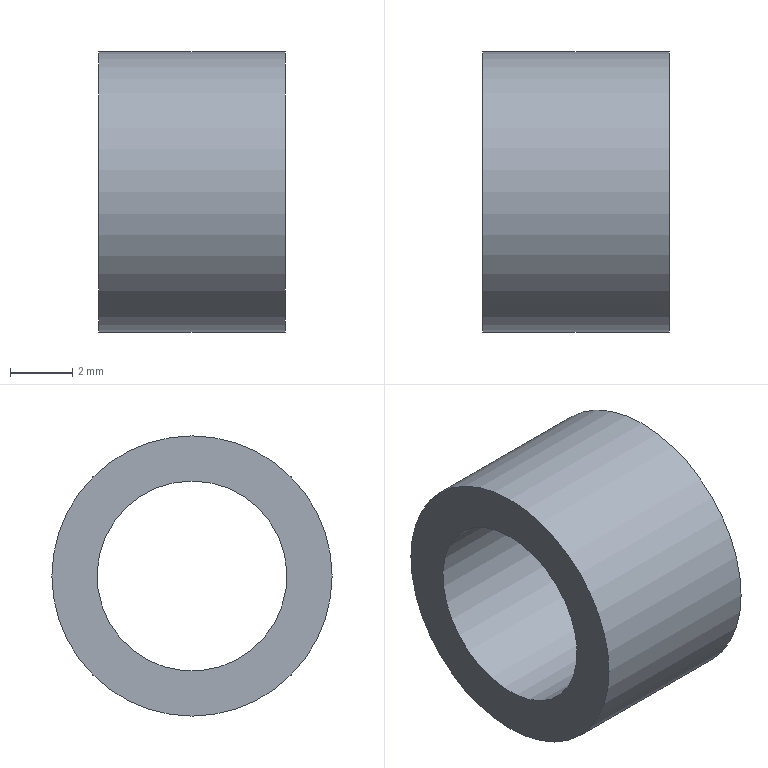Component | NX | BUSHING | 1 solid | 4 faces | box 6 x 9 x 9 mm | volume 206 mm3 | cylinder 2 | plane 2 | commonest cylinder face diameters 9 x1 6.1 x1
STEP:
#1=CARTESIAN_POINT('',(0.,0.,0.));
#2=DIRECTION('',(0.,0.,1.));
#3=DIRECTION('',(1.,0.,0.));
#4=AXIS2_PLACEMENT_3D('',#1,#2,#3);
#5=CARTESIAN_POINT('',(15.144,16.19,-72.915));
#6=VERTEX_POINT('',#5);
#7=CARTESIAN_POINT('',(15.144,16.19,-77.415));
#8=DIRECTION('',(-1.,0.,0.));
#9=DIRECTION('',(0.,0.,1.));
#10=AXIS2_PLACEMENT_3D('',#7,#8,#9);
#11=CIRCLE('',#10,4.5);
#12=CARTESIAN_POINT('',(15.144,16.19,-77.415));
#13=DIRECTION('',(1.,0.,0.));
#14=DIRECTION('',(0.,0.,-1.));
#15=AXIS2_PLACEMENT_3D('',#12,#13,#14);
#16=CYLINDRICAL_SURFACE('',#15,4.5);
#17=CARTESIAN_POINT('',(9.425,0.));
#18=DIRECTION('',(-1.,0.));
#19=VECTOR('',#18,1.);
#20=LINE('',#17,#19);
#21=(GEOMETRIC_REPRESENTATION_CONTEXT(2)PARAMETRIC_REPRESENTATION_CONTEXT()REPRESENTATION_CONTEXT('',''));
#22=DEFINITIONAL_REPRESENTATION('',(#20),#21);
#23=PCURVE('',#16,#22);
#24=CARTESIAN_POINT('',(15.144,16.19,-77.415));
#25=DIRECTION('',(-1.,0.,0.));
#26=DIRECTION('',(0.,0.,1.));
#27=AXIS2_PLACEMENT_3D('',#24,#25,#26);
#28=PLANE('',#27);
#29=CARTESIAN_POINT('',(0.,0.));
#30=DIRECTION('',(1.,0.));
#31=AXIS2_PLACEMENT_2D('',#29,#30);
#32=CIRCLE('',#31,4.5);
#33=(GEOMETRIC_REPRESENTATION_CONTEXT(2)PARAMETRIC_REPRESENTATION_CONTEXT()REPRESENTATION_CONTEXT('',''));
#34=DEFINITIONAL_REPRESENTATION('',(#32),#33);
#35=PCURVE('',#28,#34);
#36=SURFACE_CURVE('',#11,(#23,#35),.PCURVE_S1.);
#37=EDGE_CURVE('',#6,#6,#36,.T.);
#38=ORIENTED_EDGE('',*,*,#37,.F.);
#39=CARTESIAN_POINT('',(21.144,16.19,-72.915));
#40=VERTEX_POINT('',#39);
#41=CARTESIAN_POINT('',(15.144,16.19,-72.915));
#42=CARTESIAN_POINT('',(21.144,16.19,-72.915));
#43=B_SPLINE_CURVE_WITH_KNOTS('',1,(#41,#42),.UNSPECIFIED.,.F.,.F.,(2,2),(0.,6.),.PIECEWISE_BEZIER_KNOTS.);
#44=CARTESIAN_POINT('',(9.425,0.));
#45=DIRECTION('',(0.,1.));
#46=VECTOR('',#45,1.);
#47=LINE('',#44,#46);
#48=(GEOMETRIC_REPRESENTATION_CONTEXT(2)PARAMETRIC_REPRESENTATION_CONTEXT()REPRESENTATION_CONTEXT('',''));
#49=DEFINITIONAL_REPRESENTATION('',(#47),#48);
#50=PCURVE('',#16,#49);
#51=CARTESIAN_POINT('',(3.142,0.));
#52=DIRECTION('',(0.,1.));
#53=VECTOR('',#52,1.);
#54=LINE('',#51,#53);
#55=(GEOMETRIC_REPRESENTATION_CONTEXT(2)PARAMETRIC_REPRESENTATION_CONTEXT()REPRESENTATION_CONTEXT('',''));
#56=DEFINITIONAL_REPRESENTATION('',(#54),#55);
#57=PCURVE('',#16,#56);
#58=SEAM_CURVE('',#43,(#50,#57),.PCURVE_S1.);
#59=EDGE_CURVE('',#6,#40,#58,.T.);
#60=ORIENTED_EDGE('',*,*,#59,.T.);
#61=CARTESIAN_POINT('',(21.144,16.19,-77.415));
#62=DIRECTION('',(-1.,0.,0.));
#63=DIRECTION('',(0.,0.,1.));
#64=AXIS2_PLACEMENT_3D('',#61,#62,#63);
#65=CIRCLE('',#64,4.5);
#66=CARTESIAN_POINT('',(9.425,6.));
#67=DIRECTION('',(-1.,0.));
#68=VECTOR('',#67,1.);
#69=LINE('',#66,#68);
#70=(GEOMETRIC_REPRESENTATION_CONTEXT(2)PARAMETRIC_REPRESENTATION_CONTEXT()REPRESENTATION_CONTEXT('',''));
#71=DEFINITIONAL_REPRESENTATION('',(#69),#70);
#72=PCURVE('',#16,#71);
#73=CARTESIAN_POINT('',(21.144,16.19,-77.415));
#74=DIRECTION('',(-1.,0.,0.));
#75=DIRECTION('',(0.,0.,1.));
#76=AXIS2_PLACEMENT_3D('',#73,#74,#75);
#77=PLANE('',#76);
#78=CARTESIAN_POINT('',(0.,0.));
#79=DIRECTION('',(1.,0.));
#80=AXIS2_PLACEMENT_2D('',#78,#79);
#81=CIRCLE('',#80,4.5);
#82=(GEOMETRIC_REPRESENTATION_CONTEXT(2)PARAMETRIC_REPRESENTATION_CONTEXT()REPRESENTATION_CONTEXT('',''));
#83=DEFINITIONAL_REPRESENTATION('',(#81),#82);
#84=PCURVE('',#77,#83);
#85=SURFACE_CURVE('',#65,(#72,#84),.PCURVE_S1.);
#86=EDGE_CURVE('',#40,#40,#85,.T.);
#87=ORIENTED_EDGE('',*,*,#86,.T.);
#88=ORIENTED_EDGE('',*,*,#59,.F.);
#89=EDGE_LOOP('',(#38,#60,#87,#88));
#90=FACE_BOUND('',#89,.T.);
#91=ADVANCED_FACE('',(#90),#16,.T.);
#92=CARTESIAN_POINT('',(15.144,16.19,-74.365));
#93=VERTEX_POINT('',#92);
#94=CARTESIAN_POINT('',(15.144,16.19,-77.415));
#95=DIRECTION('',(-1.,0.,0.));
#96=DIRECTION('',(0.,0.,1.));
#97=AXIS2_PLACEMENT_3D('',#94,#95,#96);
#98=CIRCLE('',#97,3.05);
#99=CARTESIAN_POINT('',(15.144,16.19,-77.415));
#100=DIRECTION('',(1.,0.,0.));
#101=DIRECTION('',(0.,0.,-1.));
#102=AXIS2_PLACEMENT_3D('',#99,#100,#101);
#103=CYLINDRICAL_SURFACE('',#102,3.05);
#104=CARTESIAN_POINT('',(9.425,0.));
#105=DIRECTION('',(-1.,0.));
#106=VECTOR('',#105,1.);
#107=LINE('',#104,#106);
#108=(GEOMETRIC_REPRESENTATION_CONTEXT(2)PARAMETRIC_REPRESENTATION_CONTEXT()REPRESENTATION_CONTEXT('',''));
#109=DEFINITIONAL_REPRESENTATION('',(#107),#108);
#110=PCURVE('',#103,#109);
#111=CARTESIAN_POINT('',(0.,0.));
#112=DIRECTION('',(1.,0.));
#113=AXIS2_PLACEMENT_2D('',#111,#112);
#114=CIRCLE('',#113,3.05);
#115=(GEOMETRIC_REPRESENTATION_CONTEXT(2)PARAMETRIC_REPRESENTATION_CONTEXT()REPRESENTATION_CONTEXT('',''));
#116=DEFINITIONAL_REPRESENTATION('',(#114),#115);
#117=PCURVE('',#28,#116);
#118=SURFACE_CURVE('',#98,(#110,#117),.PCURVE_S1.);
#119=EDGE_CURVE('',#93,#93,#118,.T.);
#120=ORIENTED_EDGE('',*,*,#119,.F.);
#121=CARTESIAN_POINT('',(21.144,16.19,-74.365));
#122=VERTEX_POINT('',#121);
#123=CARTESIAN_POINT('',(15.144,16.19,-74.365));
#124=CARTESIAN_POINT('',(21.144,16.19,-74.365));
#125=B_SPLINE_CURVE_WITH_KNOTS('',1,(#123,#124),.UNSPECIFIED.,.F.,.F.,(2,2),(0.,6.),.PIECEWISE_BEZIER_KNOTS.);
#126=CARTESIAN_POINT('',(9.425,0.));
#127=DIRECTION('',(0.,1.));
#128=VECTOR('',#127,1.);
#129=LINE('',#126,#128);
#130=(GEOMETRIC_REPRESENTATION_CONTEXT(2)PARAMETRIC_REPRESENTATION_CONTEXT()REPRESENTATION_CONTEXT('',''));
#131=DEFINITIONAL_REPRESENTATION('',(#129),#130);
#132=PCURVE('',#103,#131);
#133=CARTESIAN_POINT('',(3.142,0.));
#134=DIRECTION('',(0.,1.));
#135=VECTOR('',#134,1.);
#136=LINE('',#133,#135);
#137=(GEOMETRIC_REPRESENTATION_CONTEXT(2)PARAMETRIC_REPRESENTATION_CONTEXT()REPRESENTATION_CONTEXT('',''));
#138=DEFINITIONAL_REPRESENTATION('',(#136),#137);
#139=PCURVE('',#103,#138);
#140=SEAM_CURVE('',#125,(#132,#139),.PCURVE_S1.);
#141=EDGE_CURVE('',#93,#122,#140,.T.);
#142=ORIENTED_EDGE('',*,*,#141,.T.);
#143=CARTESIAN_POINT('',(21.144,16.19,-77.415));
#144=DIRECTION('',(-1.,0.,0.));
#145=DIRECTION('',(0.,0.,1.));
#146=AXIS2_PLACEMENT_3D('',#143,#144,#145);
#147=CIRCLE('',#146,3.05);
#148=CARTESIAN_POINT('',(9.425,6.));
#149=DIRECTION('',(-1.,0.));
#150=VECTOR('',#149,1.);
#151=LINE('',#148,#150);
#152=(GEOMETRIC_REPRESENTATION_CONTEXT(2)PARAMETRIC_REPRESENTATION_CONTEXT()REPRESENTATION_CONTEXT('',''));
#153=DEFINITIONAL_REPRESENTATION('',(#151),#152);
#154=PCURVE('',#103,#153);
#155=CARTESIAN_POINT('',(0.,0.));
#156=DIRECTION('',(1.,0.));
#157=AXIS2_PLACEMENT_2D('',#155,#156);
#158=CIRCLE('',#157,3.05);
#159=(GEOMETRIC_REPRESENTATION_CONTEXT(2)PARAMETRIC_REPRESENTATION_CONTEXT()REPRESENTATION_CONTEXT('',''));
#160=DEFINITIONAL_REPRESENTATION('',(#158),#159);
#161=PCURVE('',#77,#160);
#162=SURFACE_CURVE('',#147,(#154,#161),.PCURVE_S1.);
#163=EDGE_CURVE('',#122,#122,#162,.T.);
#164=ORIENTED_EDGE('',*,*,#163,.T.);
#165=ORIENTED_EDGE('',*,*,#141,.F.);
#166=EDGE_LOOP('',(#120,#142,#164,#165));
#167=FACE_BOUND('',#166,.F.);
#168=ADVANCED_FACE('',(#167),#103,.F.);
#169=ORIENTED_EDGE('',*,*,#37,.T.);
#170=EDGE_LOOP('',(#169));
#171=FACE_BOUND('',#170,.T.);
#172=ORIENTED_EDGE('',*,*,#119,.F.);
#173=EDGE_LOOP('',(#172));
#174=FACE_BOUND('',#173,.T.);
#175=ADVANCED_FACE('',(#171,#174),#28,.T.);
#176=ORIENTED_EDGE('',*,*,#86,.F.);
#177=EDGE_LOOP('',(#176));
#178=FACE_BOUND('',#177,.T.);
#179=ORIENTED_EDGE('',*,*,#163,.T.);
#180=EDGE_LOOP('',(#179));
#181=FACE_BOUND('',#180,.T.);
#182=ADVANCED_FACE('',(#178,#181),#77,.F.);
#183=CLOSED_SHELL('',(#91,#168,#175,#182));
#184=MANIFOLD_SOLID_BREP('',#183);
#185=(LENGTH_UNIT()NAMED_UNIT(*)SI_UNIT(.MILLI.,.METRE.));
#186=UNCERTAINTY_MEASURE_WITH_UNIT(LENGTH_MEASURE(0.00001),#185,'','');
#187=(NAMED_UNIT(*)PLANE_ANGLE_UNIT()SI_UNIT($,.RADIAN.));
#188=(NAMED_UNIT(*)SI_UNIT($,.STERADIAN.)SOLID_ANGLE_UNIT());
#189=(GEOMETRIC_REPRESENTATION_CONTEXT(3)GLOBAL_UNCERTAINTY_ASSIGNED_CONTEXT((#186))GLOBAL_UNIT_ASSIGNED_CONTEXT((#185,#187,#188))REPRESENTATION_CONTEXT('',''));
#190=ADVANCED_BREP_SHAPE_REPRESENTATION('',(#4,#184),#189);